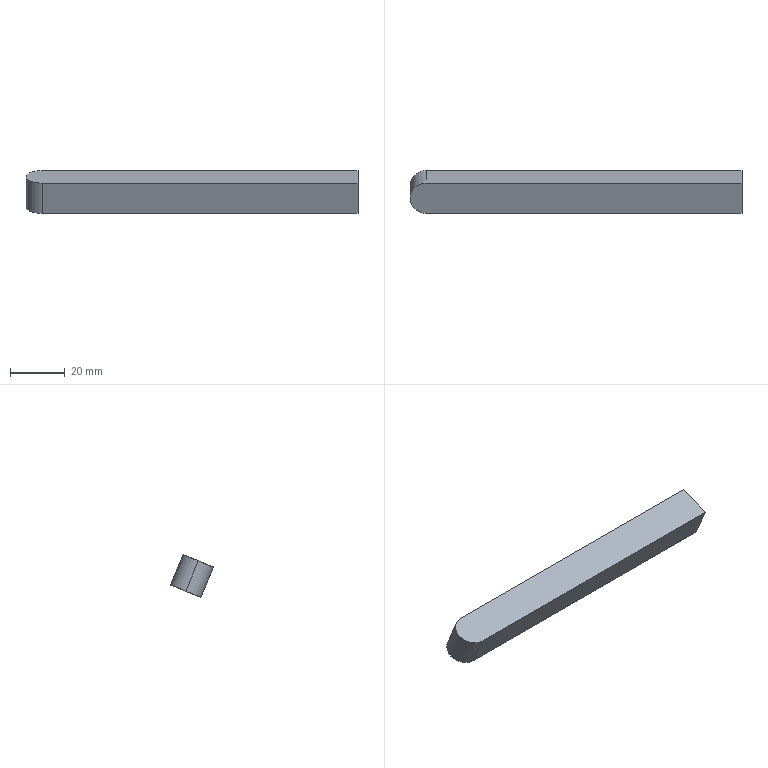Component | SolidWorks | 2026.08.03NewSchemeConnectingRod-2 | 1 solid | 11 faces | box 121.64 x 15.67 x 15.67 mm | volume 14874 mm3 | plane 5 | cylinder 4 | cone 2 | commonest cylinder face diameters 8.5 x2 12 x2
build123d program:
from build123d import *

# Parameters (mm, degrees)
BOSS_EXTRUDE1_DEPTH    = 12
M10_TAPPED_HOLE1_D     = 8.5
M10_TAPPED_HOLE1_DEPTH = 42.446
M10_TAPPED_HOLE1_TIP   = 2.554


with BuildPart() as part:
    # Sketch1 → Boss-Extrude1 (new body)
    with BuildSketch(Plane.XY):
        with BuildLine():
            Line((9.192, 6), (124.835, 6))
            Line((124.835, 6), (124.835, -6))
            Line((124.835, -6), (9.192, -6))
            ThreePointArc((9.192, -6), (3.192, 0), (9.192, 6))
        make_face()
    extrude(amount=BOSS_EXTRUDE1_DEPTH)

    # M10 Tapped Hole1
    with Locations(Plane(origin=(124.835, 0, 0), x_dir=(0, 0, -1), z_dir=(1, 0, 0))):
        with Locations((-6, 0)):
            Hole(M10_TAPPED_HOLE1_D / 2, depth=M10_TAPPED_HOLE1_DEPTH)
            with Locations((0, 0, -(M10_TAPPED_HOLE1_DEPTH + M10_TAPPED_HOLE1_TIP / 2))):  # 118° drill point
                Cone(0, M10_TAPPED_HOLE1_D / 2, M10_TAPPED_HOLE1_TIP, mode=Mode.SUBTRACT)


solid = part.part

# Placed as in the assembly
solid = solid.moved(Location((-5.641, 0.6532, 24.308), (-157.552, 0, 0)))
STEP:
#1=COLOUR_RGB('',0.7922,0.8196,0.9333);
#2=FILL_AREA_STYLE_COLOUR('',#1);
#3=FILL_AREA_STYLE('',(#2));
#4=SURFACE_STYLE_FILL_AREA(#3);
#5=SURFACE_SIDE_STYLE('',(#4));
#6=SURFACE_STYLE_USAGE(.BOTH.,#5);
#7=PRESENTATION_STYLE_ASSIGNMENT((#6));
#8=CARTESIAN_POINT('',(3.022,0.05203,0.8933));
#9=VERTEX_POINT('',#8);
#10=CARTESIAN_POINT('',(3.022,0.1798,0.584));
#11=VERTEX_POINT('',#10);
#12=CARTESIAN_POINT('',(3.022,0.1159,0.7387));
#13=DIRECTION('',(1.,0.,0.));
#14=DIRECTION('',(0.,0.3818,-0.9242));
#15=AXIS2_PLACEMENT_3D('',#12,#13,#14);
#16=CIRCLE('',#15,0.1673);
#17=EDGE_CURVE('',#9,#11,#16,.T.);
#18=ORIENTED_EDGE('',*,*,#17,.F.);
#19=CARTESIAN_POINT('',(4.693,0.05203,0.8933));
#20=VERTEX_POINT('',#19);
#21=CARTESIAN_POINT('',(4.693,0.05203,0.8933));
#22=DIRECTION('',(1.,0.,0.));
#23=VECTOR('',#22,39.37);
#24=LINE('',#21,#23);
#25=EDGE_CURVE('',#9,#20,#24,.T.);
#26=ORIENTED_EDGE('',*,*,#25,.T.);
#27=CARTESIAN_POINT('',(4.693,0.1798,0.584));
#28=VERTEX_POINT('',#27);
#29=CARTESIAN_POINT('',(4.693,0.1159,0.7387));
#30=DIRECTION('',(1.,0.,0.));
#31=DIRECTION('',(0.,0.3818,-0.9242));
#32=AXIS2_PLACEMENT_3D('',#29,#30,#31);
#33=CIRCLE('',#32,0.1673);
#34=EDGE_CURVE('',#20,#28,#33,.T.);
#35=ORIENTED_EDGE('',*,*,#34,.T.);
#36=CARTESIAN_POINT('',(4.693,0.1798,0.584));
#37=DIRECTION('',(1.,0.,0.));
#38=VECTOR('',#37,39.37);
#39=LINE('',#36,#38);
#40=EDGE_CURVE('',#11,#28,#39,.T.);
#41=ORIENTED_EDGE('',*,*,#40,.F.);
#42=EDGE_LOOP('',(#18,#26,#35,#41));
#43=FACE_OUTER_BOUND('',#42,.T.);
#44=CARTESIAN_POINT('',(4.693,0.1159,0.7387));
#45=DIRECTION('',(1.,0.,0.));
#46=DIRECTION('',(0.,0.3818,-0.9242));
#47=AXIS2_PLACEMENT_3D('',#44,#45,#46);
#48=CYLINDRICAL_SURFACE('',#47,0.1673);
#49=ADVANCED_FACE('',(#43),#48,.F.);
#50=CARTESIAN_POINT('',(2.921,0.1159,0.7387));
#51=VERTEX_POINT('',#50);
#52=CARTESIAN_POINT('',(3.022,0.1798,0.584));
#53=DIRECTION('',(0.515,0.3273,-0.7922));
#54=VECTOR('',#53,39.37);
#55=LINE('',#52,#54);
#56=EDGE_CURVE('',#51,#11,#55,.T.);
#57=ORIENTED_EDGE('',*,*,#56,.F.);
#58=CARTESIAN_POINT('',(3.022,0.05203,0.8933));
#59=DIRECTION('',(0.515,-0.3273,0.7922));
#60=VECTOR('',#59,39.37);
#61=LINE('',#58,#60);
#62=EDGE_CURVE('',#51,#9,#61,.T.);
#63=ORIENTED_EDGE('',*,*,#62,.T.);
#64=ORIENTED_EDGE('',*,*,#17,.T.);
#65=EDGE_LOOP('',(#57,#63,#64));
#66=FACE_OUTER_BOUND('',#65,.T.);
#67=CARTESIAN_POINT('',(3.022,0.1159,0.7387));
#68=DIRECTION('',(1.,0.,0.));
#69=DIRECTION('',(0.,0.3818,-0.9242));
#70=AXIS2_PLACEMENT_3D('',#67,#68,#69);
#71=CONICAL_SURFACE('',#70,0.1673,1.03);
#72=ADVANCED_FACE('',(#66),#71,.F.);
#73=CARTESIAN_POINT('',(-0.09642,0.02572,0.957));
#74=VERTEX_POINT('',#73);
#75=CARTESIAN_POINT('',(0.1398,-0.1926,0.8668));
#76=VERTEX_POINT('',#75);
#77=CARTESIAN_POINT('',(0.1398,0.02572,0.957));
#78=DIRECTION('',(-0.,-0.3818,0.9242));
#79=DIRECTION('',(1.,0.,0.));
#80=AXIS2_PLACEMENT_3D('',#77,#78,#79);
#81=CIRCLE('',#80,0.2362);
#82=EDGE_CURVE('',#74,#76,#81,.T.);
#83=ORIENTED_EDGE('',*,*,#82,.F.);
#84=CARTESIAN_POINT('',(-0.09642,0.2061,0.5204));
#85=VERTEX_POINT('',#84);
#86=CARTESIAN_POINT('',(-0.09642,0.02572,0.957));
#87=DIRECTION('',(0.,0.3818,-0.9242));
#88=VECTOR('',#87,39.37);
#89=LINE('',#86,#88);
#90=EDGE_CURVE('',#74,#85,#89,.T.);
#91=ORIENTED_EDGE('',*,*,#90,.T.);
#92=CARTESIAN_POINT('',(0.1398,-0.0122,0.4302));
#93=VERTEX_POINT('',#92);
#94=CARTESIAN_POINT('',(0.1398,0.2061,0.5204));
#95=DIRECTION('',(-0.,-0.3818,0.9242));
#96=DIRECTION('',(1.,0.,0.));
#97=AXIS2_PLACEMENT_3D('',#94,#95,#96);
#98=CIRCLE('',#97,0.2362);
#99=EDGE_CURVE('',#85,#93,#98,.T.);
#100=ORIENTED_EDGE('',*,*,#99,.T.);
#101=CARTESIAN_POINT('',(0.1398,-0.1926,0.8668));
#102=DIRECTION('',(0.,0.3818,-0.9242));
#103=VECTOR('',#102,39.37);
#104=LINE('',#101,#103);
#105=EDGE_CURVE('',#76,#93,#104,.T.);
#106=ORIENTED_EDGE('',*,*,#105,.F.);
#107=EDGE_LOOP('',(#83,#91,#100,#106));
#108=FACE_OUTER_BOUND('',#107,.T.);
#109=CARTESIAN_POINT('',(0.1398,0.02572,0.957));
#110=DIRECTION('',(0.,0.3818,-0.9242));
#111=DIRECTION('',(-1.,-0.,0.));
#112=AXIS2_PLACEMENT_3D('',#109,#110,#111);
#113=CYLINDRICAL_SURFACE('',#112,0.2362);
#114=ADVANCED_FACE('',(#108),#113,.T.);
#115=ORIENTED_EDGE('',*,*,#90,.F.);
#116=CARTESIAN_POINT('',(0.1398,0.244,1.047));
#117=VERTEX_POINT('',#116);
#118=CARTESIAN_POINT('',(0.1398,0.02572,0.957));
#119=DIRECTION('',(-0.,-0.3818,0.9242));
#120=DIRECTION('',(1.,0.,0.));
#121=AXIS2_PLACEMENT_3D('',#118,#119,#120);
#122=CIRCLE('',#121,0.2362);
#123=EDGE_CURVE('',#117,#74,#122,.T.);
#124=ORIENTED_EDGE('',*,*,#123,.F.);
#125=CARTESIAN_POINT('',(0.1398,0.4244,0.6106));
#126=VERTEX_POINT('',#125);
#127=CARTESIAN_POINT('',(0.1398,0.244,1.047));
#128=DIRECTION('',(0.,0.3818,-0.9242));
#129=VECTOR('',#128,39.37);
#130=LINE('',#127,#129);
#131=EDGE_CURVE('',#117,#126,#130,.T.);
#132=ORIENTED_EDGE('',*,*,#131,.T.);
#133=CARTESIAN_POINT('',(0.1398,0.2061,0.5204));
#134=DIRECTION('',(-0.,-0.3818,0.9242));
#135=DIRECTION('',(1.,0.,0.));
#136=AXIS2_PLACEMENT_3D('',#133,#134,#135);
#137=CIRCLE('',#136,0.2362);
#138=EDGE_CURVE('',#126,#85,#137,.T.);
#139=ORIENTED_EDGE('',*,*,#138,.T.);
#140=EDGE_LOOP('',(#115,#124,#132,#139));
#141=FACE_OUTER_BOUND('',#140,.T.);
#142=CARTESIAN_POINT('',(0.1398,0.02572,0.957));
#143=DIRECTION('',(0.,0.3818,-0.9242));
#144=DIRECTION('',(-1.,-0.,0.));
#145=AXIS2_PLACEMENT_3D('',#142,#143,#144);
#146=CYLINDRICAL_SURFACE('',#145,0.2362);
#147=ADVANCED_FACE('',(#141),#146,.T.);
#148=CARTESIAN_POINT('',(4.693,-0.0122,0.4302));
#149=VERTEX_POINT('',#148);
#150=CARTESIAN_POINT('',(0.1398,-0.0122,0.4302));
#151=DIRECTION('',(1.,0.,0.));
#152=VECTOR('',#151,39.37);
#153=LINE('',#150,#152);
#154=EDGE_CURVE('',#93,#149,#153,.T.);
#155=ORIENTED_EDGE('',*,*,#154,.T.);
#156=CARTESIAN_POINT('',(4.693,-0.1926,0.8668));
#157=VERTEX_POINT('',#156);
#158=CARTESIAN_POINT('',(4.693,-0.1926,0.8668));
#159=DIRECTION('',(0.,0.3818,-0.9242));
#160=VECTOR('',#159,39.37);
#161=LINE('',#158,#160);
#162=EDGE_CURVE('',#157,#149,#161,.T.);
#163=ORIENTED_EDGE('',*,*,#162,.F.);
#164=CARTESIAN_POINT('',(0.1398,-0.1926,0.8668));
#165=DIRECTION('',(1.,0.,0.));
#166=VECTOR('',#165,39.37);
#167=LINE('',#164,#166);
#168=EDGE_CURVE('',#76,#157,#167,.T.);
#169=ORIENTED_EDGE('',*,*,#168,.F.);
#170=ORIENTED_EDGE('',*,*,#105,.T.);
#171=EDGE_LOOP('',(#155,#163,#169,#170));
#172=FACE_OUTER_BOUND('',#171,.T.);
#173=CARTESIAN_POINT('',(0.1398,-0.1926,0.8668));
#174=DIRECTION('',(-0.,0.9242,0.3818));
#175=DIRECTION('',(-0.,-0.3818,0.9242));
#176=AXIS2_PLACEMENT_3D('',#173,#174,#175);
#177=PLANE('',#176);
#178=ADVANCED_FACE('',(#172),#177,.F.);
#179=CARTESIAN_POINT('',(4.693,0.1159,0.7387));
#180=DIRECTION('',(1.,0.,0.));
#181=DIRECTION('',(0.,0.3818,-0.9242));
#182=AXIS2_PLACEMENT_3D('',#179,#180,#181);
#183=CIRCLE('',#182,0.1673);
#184=EDGE_CURVE('',#28,#20,#183,.T.);
#185=ORIENTED_EDGE('',*,*,#184,.F.);
#186=ORIENTED_EDGE('',*,*,#34,.F.);
#187=EDGE_LOOP('',(#185,#186));
#188=FACE_BOUND('',#187,.T.);
#189=CARTESIAN_POINT('',(4.693,0.4244,0.6106));
#190=VERTEX_POINT('',#189);
#191=CARTESIAN_POINT('',(4.693,0.4244,0.6106));
#192=DIRECTION('',(-0.,0.9242,0.3818));
#193=VECTOR('',#192,39.37);
#194=LINE('',#191,#193);
#195=EDGE_CURVE('',#149,#190,#194,.T.);
#196=ORIENTED_EDGE('',*,*,#195,.T.);
#197=CARTESIAN_POINT('',(4.693,0.244,1.047));
#198=VERTEX_POINT('',#197);
#199=CARTESIAN_POINT('',(4.693,0.244,1.047));
#200=DIRECTION('',(0.,0.3818,-0.9242));
#201=VECTOR('',#200,39.37);
#202=LINE('',#199,#201);
#203=EDGE_CURVE('',#198,#190,#202,.T.);
#204=ORIENTED_EDGE('',*,*,#203,.F.);
#205=CARTESIAN_POINT('',(4.693,0.244,1.047));
#206=DIRECTION('',(-0.,0.9242,0.3818));
#207=VECTOR('',#206,39.37);
#208=LINE('',#205,#207);
#209=EDGE_CURVE('',#157,#198,#208,.T.);
#210=ORIENTED_EDGE('',*,*,#209,.F.);
#211=ORIENTED_EDGE('',*,*,#162,.T.);
#212=EDGE_LOOP('',(#196,#204,#210,#211));
#213=FACE_OUTER_BOUND('',#212,.T.);
#214=CARTESIAN_POINT('',(4.693,0.244,1.047));
#215=DIRECTION('',(-1.,-0.,-0.));
#216=DIRECTION('',(-0.,-0.3818,0.9242));
#217=AXIS2_PLACEMENT_3D('',#214,#215,#216);
#218=PLANE('',#217);
#219=ADVANCED_FACE('',(#188,#213),#218,.F.);
#220=CARTESIAN_POINT('',(0.1398,0.4244,0.6106));
#221=DIRECTION('',(-1.,-0.,-0.));
#222=VECTOR('',#221,39.37);
#223=LINE('',#220,#222);
#224=EDGE_CURVE('',#190,#126,#223,.T.);
#225=ORIENTED_EDGE('',*,*,#224,.T.);
#226=ORIENTED_EDGE('',*,*,#131,.F.);
#227=CARTESIAN_POINT('',(0.1398,0.244,1.047));
#228=DIRECTION('',(-1.,-0.,-0.));
#229=VECTOR('',#228,39.37);
#230=LINE('',#227,#229);
#231=EDGE_CURVE('',#198,#117,#230,.T.);
#232=ORIENTED_EDGE('',*,*,#231,.F.);
#233=ORIENTED_EDGE('',*,*,#203,.T.);
#234=EDGE_LOOP('',(#225,#226,#232,#233));
#235=FACE_OUTER_BOUND('',#234,.T.);
#236=CARTESIAN_POINT('',(0.1398,0.244,1.047));
#237=DIRECTION('',(0.,-0.9242,-0.3818));
#238=DIRECTION('',(0.,0.3818,-0.9242));
#239=AXIS2_PLACEMENT_3D('',#236,#237,#238);
#240=PLANE('',#239);
#241=ADVANCED_FACE('',(#235),#240,.F.);
#242=ORIENTED_EDGE('',*,*,#123,.T.);
#243=ORIENTED_EDGE('',*,*,#82,.T.);
#244=ORIENTED_EDGE('',*,*,#168,.T.);
#245=ORIENTED_EDGE('',*,*,#209,.T.);
#246=ORIENTED_EDGE('',*,*,#231,.T.);
#247=EDGE_LOOP('',(#242,#243,#244,#245,#246));
#248=FACE_OUTER_BOUND('',#247,.T.);
#249=CARTESIAN_POINT('',(0.1398,0.02572,0.957));
#250=DIRECTION('',(-0.,-0.3818,0.9242));
#251=DIRECTION('',(1.,0.,0.));
#252=AXIS2_PLACEMENT_3D('',#249,#250,#251);
#253=PLANE('',#252);
#254=ADVANCED_FACE('',(#248),#253,.T.);
#255=ORIENTED_EDGE('',*,*,#138,.F.);
#256=ORIENTED_EDGE('',*,*,#224,.F.);
#257=ORIENTED_EDGE('',*,*,#195,.F.);
#258=ORIENTED_EDGE('',*,*,#154,.F.);
#259=ORIENTED_EDGE('',*,*,#99,.F.);
#260=EDGE_LOOP('',(#255,#256,#257,#258,#259));
#261=FACE_OUTER_BOUND('',#260,.T.);
#262=CARTESIAN_POINT('',(0.1398,0.2061,0.5204));
#263=DIRECTION('',(-0.,-0.3818,0.9242));
#264=DIRECTION('',(1.,0.,0.));
#265=AXIS2_PLACEMENT_3D('',#262,#263,#264);
#266=PLANE('',#265);
#267=ADVANCED_FACE('',(#261),#266,.F.);
#268=ORIENTED_EDGE('',*,*,#62,.F.);
#269=ORIENTED_EDGE('',*,*,#56,.T.);
#270=CARTESIAN_POINT('',(3.022,0.1159,0.7387));
#271=DIRECTION('',(1.,0.,0.));
#272=DIRECTION('',(0.,0.3818,-0.9242));
#273=AXIS2_PLACEMENT_3D('',#270,#271,#272);
#274=CIRCLE('',#273,0.1673);
#275=EDGE_CURVE('',#11,#9,#274,.T.);
#276=ORIENTED_EDGE('',*,*,#275,.T.);
#277=EDGE_LOOP('',(#268,#269,#276));
#278=FACE_OUTER_BOUND('',#277,.T.);
#279=CARTESIAN_POINT('',(3.022,0.1159,0.7387));
#280=DIRECTION('',(1.,0.,0.));
#281=DIRECTION('',(0.,0.3818,-0.9242));
#282=AXIS2_PLACEMENT_3D('',#279,#280,#281);
#283=CONICAL_SURFACE('',#282,0.1673,1.03);
#284=ADVANCED_FACE('',(#278),#283,.F.);
#285=ORIENTED_EDGE('',*,*,#25,.F.);
#286=ORIENTED_EDGE('',*,*,#275,.F.);
#287=ORIENTED_EDGE('',*,*,#40,.T.);
#288=ORIENTED_EDGE('',*,*,#184,.T.);
#289=EDGE_LOOP('',(#285,#286,#287,#288));
#290=FACE_OUTER_BOUND('',#289,.T.);
#291=CARTESIAN_POINT('',(4.693,0.1159,0.7387));
#292=DIRECTION('',(1.,0.,0.));
#293=DIRECTION('',(0.,0.3818,-0.9242));
#294=AXIS2_PLACEMENT_3D('',#291,#292,#293);
#295=CYLINDRICAL_SURFACE('',#294,0.1673);
#296=ADVANCED_FACE('',(#290),#295,.F.);
#297=CLOSED_SHELL('',(#49,#72,#114,#147,#178,#219,#241,#254,#267,#284,#296));
#298=MANIFOLD_SOLID_BREP('',#297);
#299=STYLED_ITEM('',(#7),#298);
#300=(LENGTH_UNIT()NAMED_UNIT(*)SI_UNIT($,.METRE.));
#301=LENGTH_MEASURE_WITH_UNIT(LENGTH_MEASURE(0.0254),#300);
#302=DIMENSIONAL_EXPONENTS(1.,0.,0.,0.,0.,0.,0.);
#303=(CONVERSION_BASED_UNIT('',#301)LENGTH_UNIT()NAMED_UNIT(#302));
#304=UNCERTAINTY_MEASURE_WITH_UNIT(LENGTH_MEASURE(0.00001),#303,'','');
#305=(NAMED_UNIT(*)PLANE_ANGLE_UNIT()SI_UNIT($,.RADIAN.));
#306=(NAMED_UNIT(*)SI_UNIT($,.STERADIAN.)SOLID_ANGLE_UNIT());
#307=(GEOMETRIC_REPRESENTATION_CONTEXT(3)GLOBAL_UNCERTAINTY_ASSIGNED_CONTEXT((#304))GLOBAL_UNIT_ASSIGNED_CONTEXT((#303,#305,#306))REPRESENTATION_CONTEXT('',''));
#308=MECHANICAL_DESIGN_GEOMETRIC_PRESENTATION_REPRESENTATION('',(#299),#307);
#309=CARTESIAN_POINT('',(0.,0.,0.));
#310=DIRECTION('',(0.,0.,1.));
#311=DIRECTION('',(1.,0.,0.));
#312=AXIS2_PLACEMENT_3D('',#309,#310,#311);
#313=(LENGTH_UNIT()NAMED_UNIT(*)SI_UNIT($,.METRE.));
#314=LENGTH_MEASURE_WITH_UNIT(LENGTH_MEASURE(0.0254),#313);
#315=DIMENSIONAL_EXPONENTS(1.,0.,0.,0.,0.,0.,0.);
#316=(CONVERSION_BASED_UNIT('',#314)LENGTH_UNIT()NAMED_UNIT(#315));
#317=UNCERTAINTY_MEASURE_WITH_UNIT(LENGTH_MEASURE(0.00001),#316,'','');
#318=(NAMED_UNIT(*)PLANE_ANGLE_UNIT()SI_UNIT($,.RADIAN.));
#319=(NAMED_UNIT(*)SI_UNIT($,.STERADIAN.)SOLID_ANGLE_UNIT());
#320=(GEOMETRIC_REPRESENTATION_CONTEXT(3)GLOBAL_UNCERTAINTY_ASSIGNED_CONTEXT((#317))GLOBAL_UNIT_ASSIGNED_CONTEXT((#316,#318,#319))REPRESENTATION_CONTEXT('',''));
#321=ADVANCED_BREP_SHAPE_REPRESENTATION('',(#298,#312),#320);
#322=PRESENTATION_LAYER_ASSIGNMENT('','',(#299));